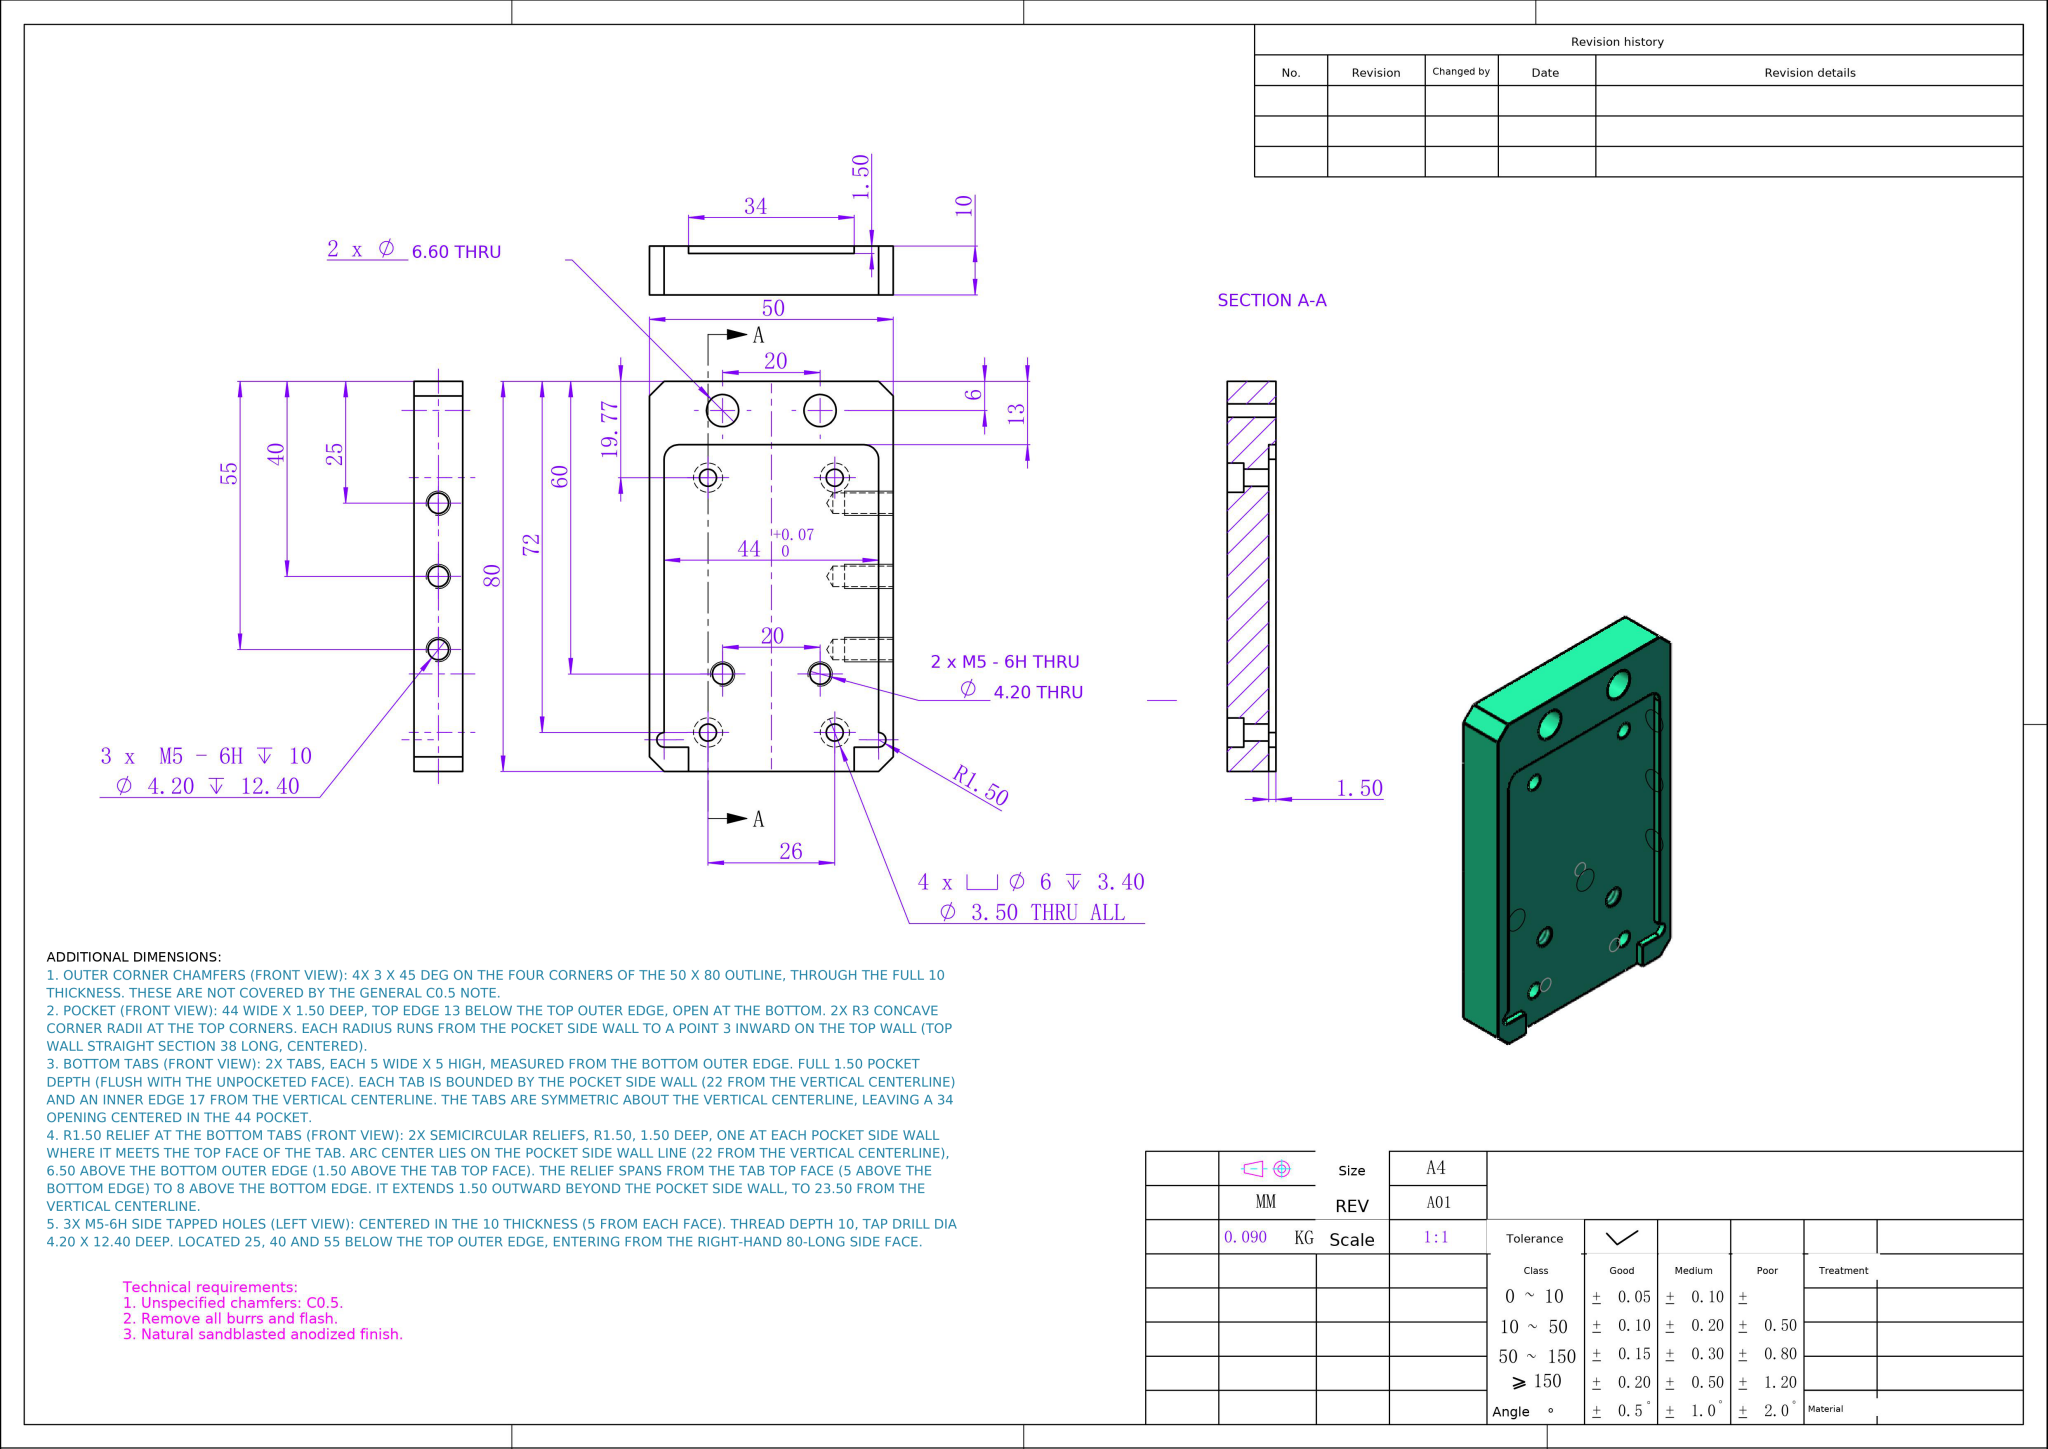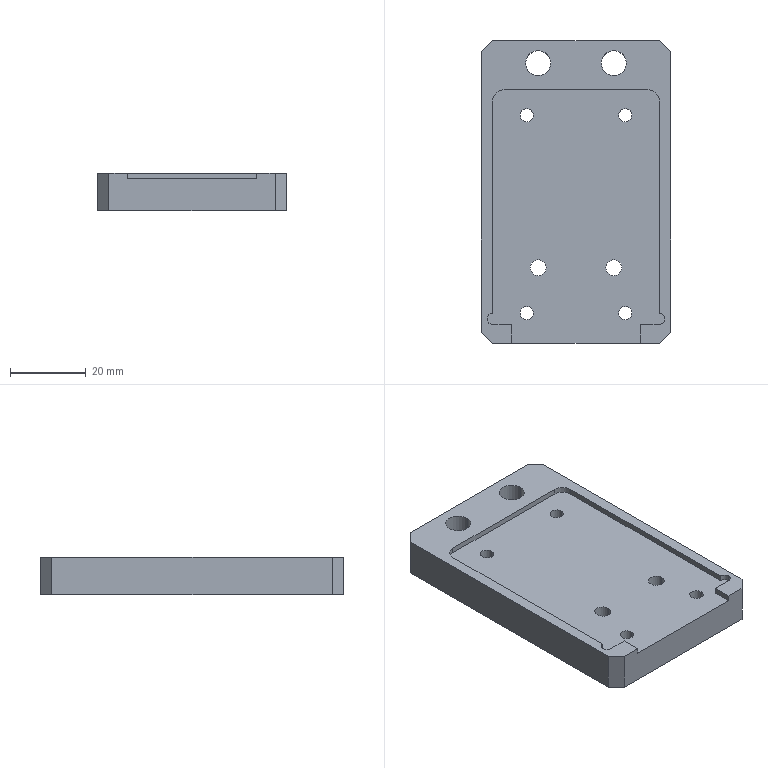Part | NX | mm | 1 solid | 63 faces | box 50 x 80 x 10 mm | volume 33435 mm3 | cylinder 35 | plane 22 | cone 6 | commonest cylinder face diameters 4.2 x10 6 x10 3.5 x8 6.6 x4 3 x3